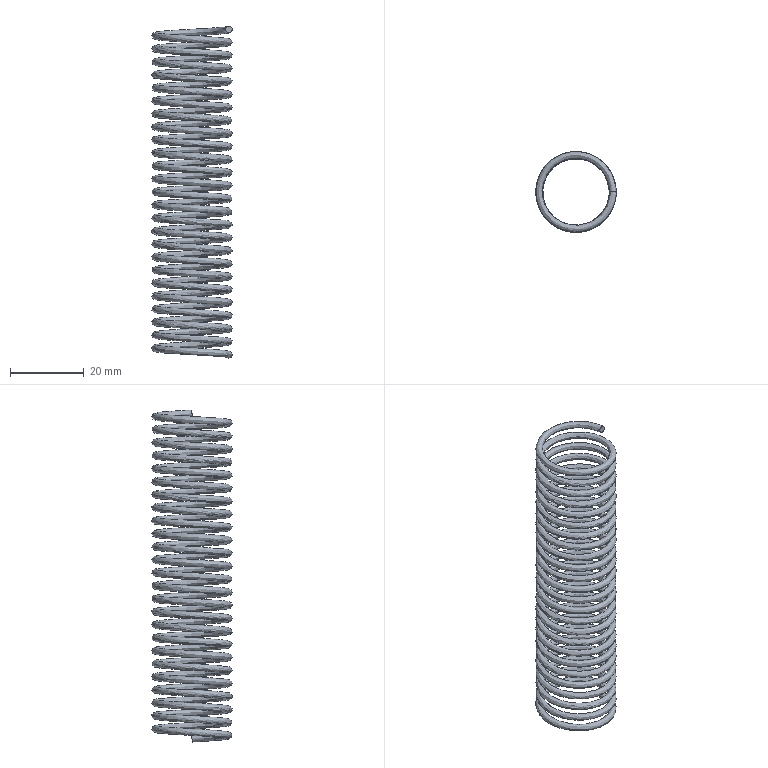Component | NX | SPRING | 1 solid | 3 faces | volume 3937 mm3 | plane 2 | spline 1